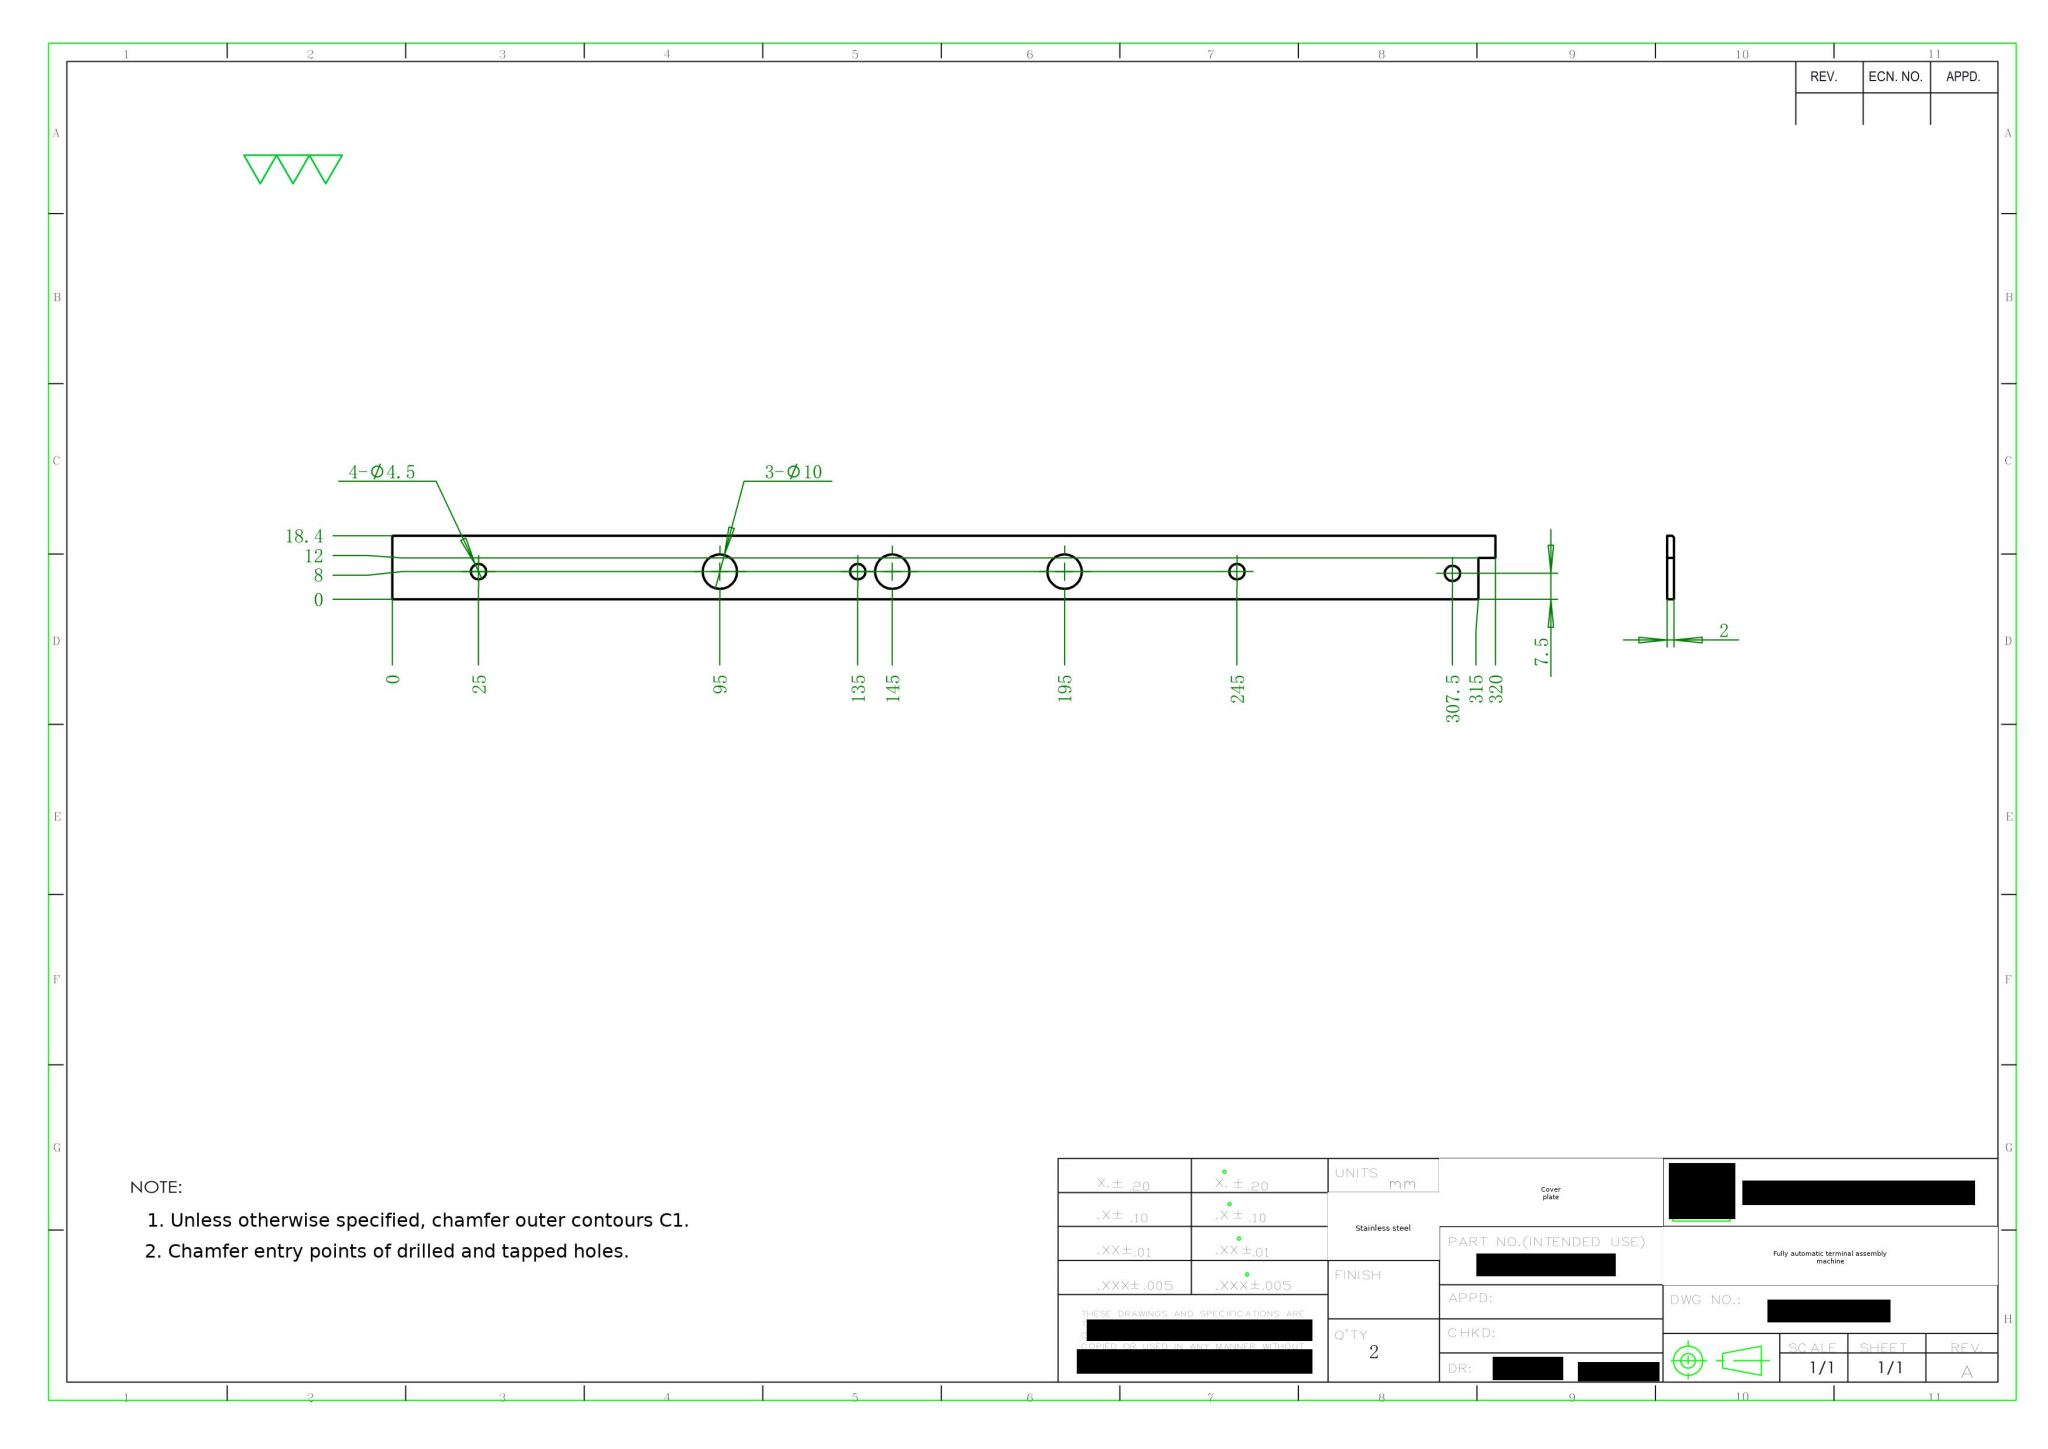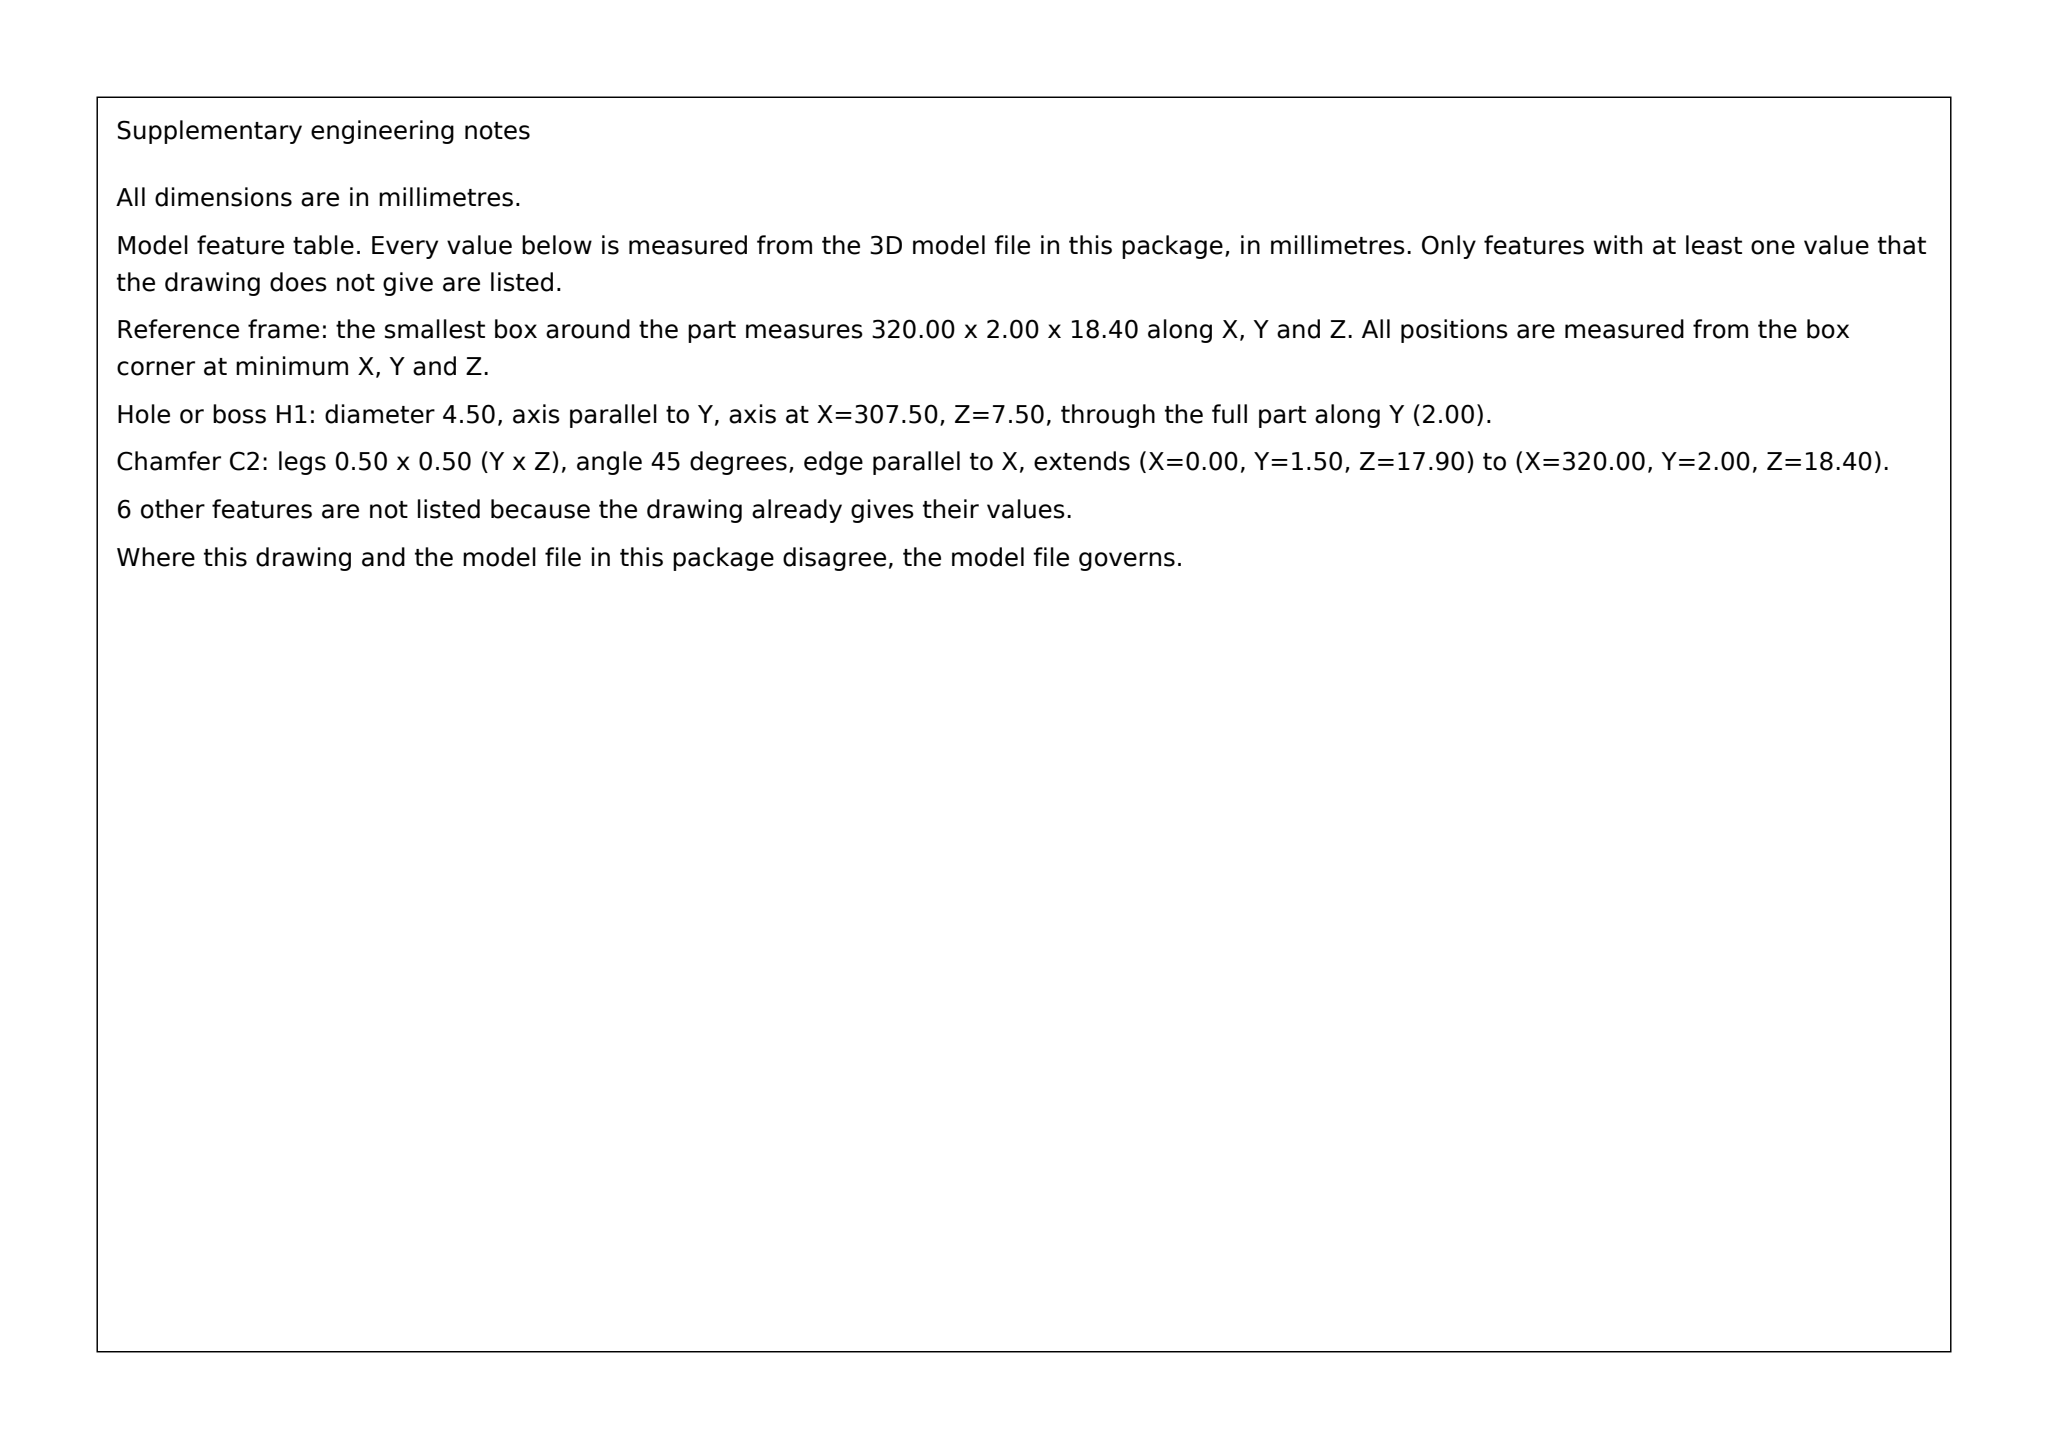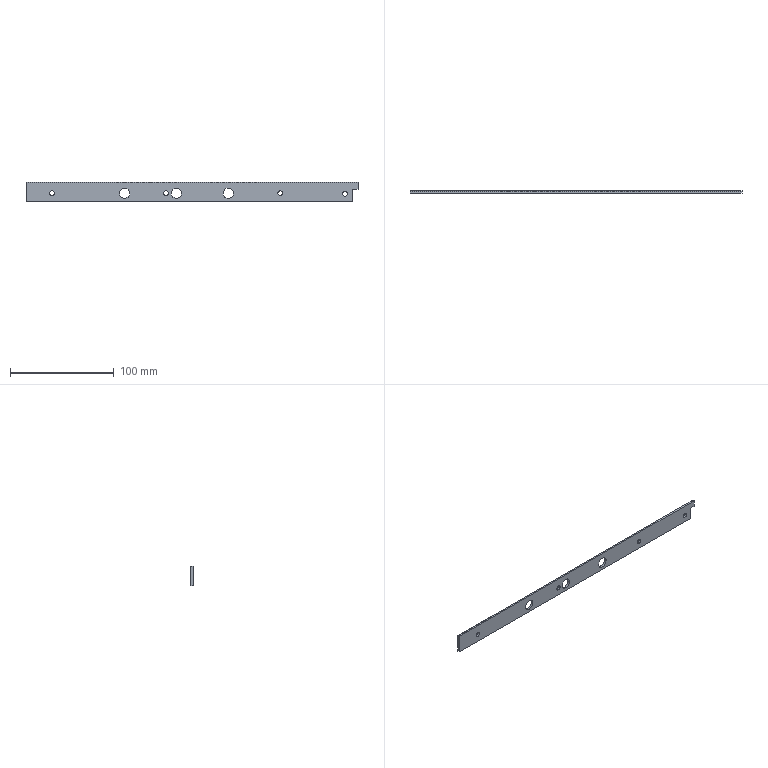Part | SolidWorks | mm | material Stainless steel | 1 solid | 23 faces | box 320 x 2 x 18.4 mm | volume 11018 mm3 | cylinder 14 | plane 9 | commonest cylinder face diameters 4.5 x8 10 x6
build123d program:
from build123d import *

# Parameters (mm, degrees)
SKETCH2_W                  = 320
SKETCH2_H                  = 18.4
BOSS_EXTRUDE1_DEPTH        = 2
CHAMFER1_SIZE              = 0.5
SKETCH8_W                  = 5
SKETCH8_H                  = 12
CUT_EXTRUDE2_DEPTH         = 161.277
F_4_5_4_5_DIAMETER_HOLE1_D = 4.5
F_10_0_10_DIAMETER_HOLE1_D = 10
F_4_5_4_5_DIAMETER_HOLE2_D = 4.5


with BuildPart() as part:
    # Sketch2 → Boss-Extrude1 (new body)
    with BuildSketch(Plane(origin=(0, 0, 0), x_dir=(1, 0, 0), z_dir=(0, 1, 0))):
        Rectangle(SKETCH2_W, SKETCH2_H)
    extrude(amount=BOSS_EXTRUDE1_DEPTH)

    # Chamfer1
    chamfer1_edges = [part.edges().sort_by_distance(p)[0] for p in [
        (0, 2, 9.2),
    ]]
    chamfer(chamfer1_edges, length=CHAMFER1_SIZE)

    # Sketch8 → Cut-Extrude2 (cut, through all)
    with BuildSketch(Plane(origin=(0, 2, 0), x_dir=(1, 0, 0), z_dir=(0, 1, 0))):
        with Locations((157.5, 3.2)):
            Rectangle(SKETCH8_W, SKETCH8_H)
    extrude(amount=-CUT_EXTRUDE2_DEPTH, mode=Mode.SUBTRACT)

    # 4.5 _4.5_ Diameter Hole1 (through all)
    with Locations(Plane(origin=(0, 2, 0), x_dir=(1, 0, 0), z_dir=(0, 1, 0))):
        with Locations((147.5, 1.7)):
            Hole(F_4_5_4_5_DIAMETER_HOLE1_D / 2)

    # 10.0 _10_ Diameter Hole1 (through all)
    with Locations(Plane(origin=(0, 2, 0), x_dir=(1, 0, 0), z_dir=(0, 1, 0))):
        with Locations((35, 1.2), (-15, 1.2), (-65, 1.2)):
            Hole(F_10_0_10_DIAMETER_HOLE1_D / 2)

    # 4.5 _4.5_ Diameter Hole2 (through all)
    with Locations(Plane(origin=(0, 0, 0), x_dir=(-1, 0, 0), z_dir=(0, -1, 0))):
        with Locations((135, 1.2), (25, 1.2), (-85, 1.2)):
            Hole(F_4_5_4_5_DIAMETER_HOLE2_D / 2)


solid = part.part
STEP:
#1=CARTESIAN_POINT('',(-135.,2.,1.05));
#2=VERTEX_POINT('',#1);
#3=CARTESIAN_POINT('',(-135.,2.,-3.45));
#4=VERTEX_POINT('',#3);
#5=CARTESIAN_POINT('',(-135.,2.,-1.2));
#6=DIRECTION('',(0.,-1.,0.));
#7=DIRECTION('',(0.,0.,-1.));
#8=AXIS2_PLACEMENT_3D('',#5,#6,#7);
#9=CIRCLE('',#8,2.25);
#10=EDGE_CURVE('',#2,#4,#9,.T.);
#11=ORIENTED_EDGE('',*,*,#10,.F.);
#12=CARTESIAN_POINT('',(-135.,0.,1.05));
#13=VERTEX_POINT('',#12);
#14=CARTESIAN_POINT('',(-135.,0.,1.05));
#15=DIRECTION('',(0.,-1.,0.));
#16=VECTOR('',#15,1000.);
#17=LINE('',#14,#16);
#18=EDGE_CURVE('',#2,#13,#17,.T.);
#19=ORIENTED_EDGE('',*,*,#18,.T.);
#20=CARTESIAN_POINT('',(-135.,0.,-3.45));
#21=VERTEX_POINT('',#20);
#22=CARTESIAN_POINT('',(-135.,0.,-1.2));
#23=DIRECTION('',(0.,-1.,0.));
#24=DIRECTION('',(0.,0.,-1.));
#25=AXIS2_PLACEMENT_3D('',#22,#23,#24);
#26=CIRCLE('',#25,2.25);
#27=EDGE_CURVE('',#13,#21,#26,.T.);
#28=ORIENTED_EDGE('',*,*,#27,.T.);
#29=CARTESIAN_POINT('',(-135.,0.,-3.45));
#30=DIRECTION('',(0.,-1.,0.));
#31=VECTOR('',#30,1000.);
#32=LINE('',#29,#31);
#33=EDGE_CURVE('',#4,#21,#32,.T.);
#34=ORIENTED_EDGE('',*,*,#33,.F.);
#35=EDGE_LOOP('',(#11,#19,#28,#34));
#36=FACE_OUTER_BOUND('',#35,.T.);
#37=CARTESIAN_POINT('',(-135.,0.,-1.2));
#38=DIRECTION('',(0.,-1.,0.));
#39=DIRECTION('',(0.,0.,-1.));
#40=AXIS2_PLACEMENT_3D('',#37,#38,#39);
#41=CYLINDRICAL_SURFACE('',#40,2.25);
#42=ADVANCED_FACE('',(#36),#41,.F.);
#43=CARTESIAN_POINT('',(-25.,2.,1.05));
#44=VERTEX_POINT('',#43);
#45=CARTESIAN_POINT('',(-25.,2.,-3.45));
#46=VERTEX_POINT('',#45);
#47=CARTESIAN_POINT('',(-25.,2.,-1.2));
#48=DIRECTION('',(0.,-1.,0.));
#49=DIRECTION('',(0.,0.,-1.));
#50=AXIS2_PLACEMENT_3D('',#47,#48,#49);
#51=CIRCLE('',#50,2.25);
#52=EDGE_CURVE('',#44,#46,#51,.T.);
#53=ORIENTED_EDGE('',*,*,#52,.F.);
#54=CARTESIAN_POINT('',(-25.,0.,1.05));
#55=VERTEX_POINT('',#54);
#56=CARTESIAN_POINT('',(-25.,0.,1.05));
#57=DIRECTION('',(0.,-1.,0.));
#58=VECTOR('',#57,1000.);
#59=LINE('',#56,#58);
#60=EDGE_CURVE('',#44,#55,#59,.T.);
#61=ORIENTED_EDGE('',*,*,#60,.T.);
#62=CARTESIAN_POINT('',(-25.,0.,-3.45));
#63=VERTEX_POINT('',#62);
#64=CARTESIAN_POINT('',(-25.,0.,-1.2));
#65=DIRECTION('',(0.,-1.,0.));
#66=DIRECTION('',(0.,0.,-1.));
#67=AXIS2_PLACEMENT_3D('',#64,#65,#66);
#68=CIRCLE('',#67,2.25);
#69=EDGE_CURVE('',#55,#63,#68,.T.);
#70=ORIENTED_EDGE('',*,*,#69,.T.);
#71=CARTESIAN_POINT('',(-25.,0.,-3.45));
#72=DIRECTION('',(0.,-1.,0.));
#73=VECTOR('',#72,1000.);
#74=LINE('',#71,#73);
#75=EDGE_CURVE('',#46,#63,#74,.T.);
#76=ORIENTED_EDGE('',*,*,#75,.F.);
#77=EDGE_LOOP('',(#53,#61,#70,#76));
#78=FACE_OUTER_BOUND('',#77,.T.);
#79=CARTESIAN_POINT('',(-25.,0.,-1.2));
#80=DIRECTION('',(0.,-1.,0.));
#81=DIRECTION('',(0.,0.,-1.));
#82=AXIS2_PLACEMENT_3D('',#79,#80,#81);
#83=CYLINDRICAL_SURFACE('',#82,2.25);
#84=ADVANCED_FACE('',(#78),#83,.F.);
#85=CARTESIAN_POINT('',(85.,2.,1.05));
#86=VERTEX_POINT('',#85);
#87=CARTESIAN_POINT('',(85.,2.,-3.45));
#88=VERTEX_POINT('',#87);
#89=CARTESIAN_POINT('',(85.,2.,-1.2));
#90=DIRECTION('',(0.,-1.,0.));
#91=DIRECTION('',(0.,0.,-1.));
#92=AXIS2_PLACEMENT_3D('',#89,#90,#91);
#93=CIRCLE('',#92,2.25);
#94=EDGE_CURVE('',#86,#88,#93,.T.);
#95=ORIENTED_EDGE('',*,*,#94,.F.);
#96=CARTESIAN_POINT('',(85.,0.,1.05));
#97=VERTEX_POINT('',#96);
#98=CARTESIAN_POINT('',(85.,0.,1.05));
#99=DIRECTION('',(0.,-1.,0.));
#100=VECTOR('',#99,1000.);
#101=LINE('',#98,#100);
#102=EDGE_CURVE('',#86,#97,#101,.T.);
#103=ORIENTED_EDGE('',*,*,#102,.T.);
#104=CARTESIAN_POINT('',(85.,0.,-3.45));
#105=VERTEX_POINT('',#104);
#106=CARTESIAN_POINT('',(85.,0.,-1.2));
#107=DIRECTION('',(0.,-1.,0.));
#108=DIRECTION('',(0.,0.,-1.));
#109=AXIS2_PLACEMENT_3D('',#106,#107,#108);
#110=CIRCLE('',#109,2.25);
#111=EDGE_CURVE('',#97,#105,#110,.T.);
#112=ORIENTED_EDGE('',*,*,#111,.T.);
#113=CARTESIAN_POINT('',(85.,0.,-3.45));
#114=DIRECTION('',(0.,-1.,0.));
#115=VECTOR('',#114,1000.);
#116=LINE('',#113,#115);
#117=EDGE_CURVE('',#88,#105,#116,.T.);
#118=ORIENTED_EDGE('',*,*,#117,.F.);
#119=EDGE_LOOP('',(#95,#103,#112,#118));
#120=FACE_OUTER_BOUND('',#119,.T.);
#121=CARTESIAN_POINT('',(85.,0.,-1.2));
#122=DIRECTION('',(0.,-1.,0.));
#123=DIRECTION('',(0.,0.,-1.));
#124=AXIS2_PLACEMENT_3D('',#121,#122,#123);
#125=CYLINDRICAL_SURFACE('',#124,2.25);
#126=ADVANCED_FACE('',(#120),#125,.F.);
#127=CARTESIAN_POINT('',(35.,0.,-6.2));
#128=VERTEX_POINT('',#127);
#129=CARTESIAN_POINT('',(35.,0.,3.8));
#130=VERTEX_POINT('',#129);
#131=CARTESIAN_POINT('',(35.,0.,-1.2));
#132=DIRECTION('',(0.,1.,0.));
#133=DIRECTION('',(0.,0.,1.));
#134=AXIS2_PLACEMENT_3D('',#131,#132,#133);
#135=CIRCLE('',#134,5.);
#136=EDGE_CURVE('',#128,#130,#135,.T.);
#137=ORIENTED_EDGE('',*,*,#136,.F.);
#138=CARTESIAN_POINT('',(35.,2.,-6.2));
#139=VERTEX_POINT('',#138);
#140=CARTESIAN_POINT('',(35.,2.,-6.2));
#141=DIRECTION('',(0.,1.,0.));
#142=VECTOR('',#141,1000.);
#143=LINE('',#140,#142);
#144=EDGE_CURVE('',#128,#139,#143,.T.);
#145=ORIENTED_EDGE('',*,*,#144,.T.);
#146=CARTESIAN_POINT('',(35.,2.,3.8));
#147=VERTEX_POINT('',#146);
#148=CARTESIAN_POINT('',(35.,2.,-1.2));
#149=DIRECTION('',(0.,1.,0.));
#150=DIRECTION('',(0.,0.,1.));
#151=AXIS2_PLACEMENT_3D('',#148,#149,#150);
#152=CIRCLE('',#151,5.);
#153=EDGE_CURVE('',#139,#147,#152,.T.);
#154=ORIENTED_EDGE('',*,*,#153,.T.);
#155=CARTESIAN_POINT('',(35.,2.,3.8));
#156=DIRECTION('',(0.,1.,0.));
#157=VECTOR('',#156,1000.);
#158=LINE('',#155,#157);
#159=EDGE_CURVE('',#130,#147,#158,.T.);
#160=ORIENTED_EDGE('',*,*,#159,.F.);
#161=EDGE_LOOP('',(#137,#145,#154,#160));
#162=FACE_OUTER_BOUND('',#161,.T.);
#163=CARTESIAN_POINT('',(35.,2.,-1.2));
#164=DIRECTION('',(0.,1.,0.));
#165=DIRECTION('',(0.,0.,1.));
#166=AXIS2_PLACEMENT_3D('',#163,#164,#165);
#167=CYLINDRICAL_SURFACE('',#166,5.);
#168=ADVANCED_FACE('',(#162),#167,.F.);
#169=CARTESIAN_POINT('',(-15.,0.,-6.2));
#170=VERTEX_POINT('',#169);
#171=CARTESIAN_POINT('',(-15.,0.,3.8));
#172=VERTEX_POINT('',#171);
#173=CARTESIAN_POINT('',(-15.,0.,-1.2));
#174=DIRECTION('',(0.,1.,0.));
#175=DIRECTION('',(0.,0.,1.));
#176=AXIS2_PLACEMENT_3D('',#173,#174,#175);
#177=CIRCLE('',#176,5.);
#178=EDGE_CURVE('',#170,#172,#177,.T.);
#179=ORIENTED_EDGE('',*,*,#178,.F.);
#180=CARTESIAN_POINT('',(-15.,2.,-6.2));
#181=VERTEX_POINT('',#180);
#182=CARTESIAN_POINT('',(-15.,2.,-6.2));
#183=DIRECTION('',(0.,1.,0.));
#184=VECTOR('',#183,1000.);
#185=LINE('',#182,#184);
#186=EDGE_CURVE('',#170,#181,#185,.T.);
#187=ORIENTED_EDGE('',*,*,#186,.T.);
#188=CARTESIAN_POINT('',(-15.,2.,3.8));
#189=VERTEX_POINT('',#188);
#190=CARTESIAN_POINT('',(-15.,2.,-1.2));
#191=DIRECTION('',(0.,1.,0.));
#192=DIRECTION('',(0.,0.,1.));
#193=AXIS2_PLACEMENT_3D('',#190,#191,#192);
#194=CIRCLE('',#193,5.);
#195=EDGE_CURVE('',#181,#189,#194,.T.);
#196=ORIENTED_EDGE('',*,*,#195,.T.);
#197=CARTESIAN_POINT('',(-15.,2.,3.8));
#198=DIRECTION('',(0.,1.,0.));
#199=VECTOR('',#198,1000.);
#200=LINE('',#197,#199);
#201=EDGE_CURVE('',#172,#189,#200,.T.);
#202=ORIENTED_EDGE('',*,*,#201,.F.);
#203=EDGE_LOOP('',(#179,#187,#196,#202));
#204=FACE_OUTER_BOUND('',#203,.T.);
#205=CARTESIAN_POINT('',(-15.,2.,-1.2));
#206=DIRECTION('',(0.,1.,0.));
#207=DIRECTION('',(0.,0.,1.));
#208=AXIS2_PLACEMENT_3D('',#205,#206,#207);
#209=CYLINDRICAL_SURFACE('',#208,5.);
#210=ADVANCED_FACE('',(#204),#209,.F.);
#211=CARTESIAN_POINT('',(-65.,0.,-6.2));
#212=VERTEX_POINT('',#211);
#213=CARTESIAN_POINT('',(-65.,0.,3.8));
#214=VERTEX_POINT('',#213);
#215=CARTESIAN_POINT('',(-65.,0.,-1.2));
#216=DIRECTION('',(0.,1.,0.));
#217=DIRECTION('',(0.,0.,1.));
#218=AXIS2_PLACEMENT_3D('',#215,#216,#217);
#219=CIRCLE('',#218,5.);
#220=EDGE_CURVE('',#212,#214,#219,.T.);
#221=ORIENTED_EDGE('',*,*,#220,.F.);
#222=CARTESIAN_POINT('',(-65.,2.,-6.2));
#223=VERTEX_POINT('',#222);
#224=CARTESIAN_POINT('',(-65.,2.,-6.2));
#225=DIRECTION('',(0.,1.,0.));
#226=VECTOR('',#225,1000.);
#227=LINE('',#224,#226);
#228=EDGE_CURVE('',#212,#223,#227,.T.);
#229=ORIENTED_EDGE('',*,*,#228,.T.);
#230=CARTESIAN_POINT('',(-65.,2.,3.8));
#231=VERTEX_POINT('',#230);
#232=CARTESIAN_POINT('',(-65.,2.,-1.2));
#233=DIRECTION('',(0.,1.,0.));
#234=DIRECTION('',(0.,0.,1.));
#235=AXIS2_PLACEMENT_3D('',#232,#233,#234);
#236=CIRCLE('',#235,5.);
#237=EDGE_CURVE('',#223,#231,#236,.T.);
#238=ORIENTED_EDGE('',*,*,#237,.T.);
#239=CARTESIAN_POINT('',(-65.,2.,3.8));
#240=DIRECTION('',(0.,1.,0.));
#241=VECTOR('',#240,1000.);
#242=LINE('',#239,#241);
#243=EDGE_CURVE('',#214,#231,#242,.T.);
#244=ORIENTED_EDGE('',*,*,#243,.F.);
#245=EDGE_LOOP('',(#221,#229,#238,#244));
#246=FACE_OUTER_BOUND('',#245,.T.);
#247=CARTESIAN_POINT('',(-65.,2.,-1.2));
#248=DIRECTION('',(0.,1.,0.));
#249=DIRECTION('',(0.,0.,1.));
#250=AXIS2_PLACEMENT_3D('',#247,#248,#249);
#251=CYLINDRICAL_SURFACE('',#250,5.);
#252=ADVANCED_FACE('',(#246),#251,.F.);
#253=CARTESIAN_POINT('',(147.5,0.,-3.95));
#254=VERTEX_POINT('',#253);
#255=CARTESIAN_POINT('',(147.5,0.,0.55));
#256=VERTEX_POINT('',#255);
#257=CARTESIAN_POINT('',(147.5,0.,-1.7));
#258=DIRECTION('',(0.,1.,0.));
#259=DIRECTION('',(0.,0.,1.));
#260=AXIS2_PLACEMENT_3D('',#257,#258,#259);
#261=CIRCLE('',#260,2.25);
#262=EDGE_CURVE('',#254,#256,#261,.T.);
#263=ORIENTED_EDGE('',*,*,#262,.F.);
#264=CARTESIAN_POINT('',(147.5,2.,-3.95));
#265=VERTEX_POINT('',#264);
#266=CARTESIAN_POINT('',(147.5,2.,-3.95));
#267=DIRECTION('',(0.,1.,0.));
#268=VECTOR('',#267,1000.);
#269=LINE('',#266,#268);
#270=EDGE_CURVE('',#254,#265,#269,.T.);
#271=ORIENTED_EDGE('',*,*,#270,.T.);
#272=CARTESIAN_POINT('',(147.5,2.,0.55));
#273=VERTEX_POINT('',#272);
#274=CARTESIAN_POINT('',(147.5,2.,-1.7));
#275=DIRECTION('',(0.,1.,0.));
#276=DIRECTION('',(0.,0.,1.));
#277=AXIS2_PLACEMENT_3D('',#274,#275,#276);
#278=CIRCLE('',#277,2.25);
#279=EDGE_CURVE('',#265,#273,#278,.T.);
#280=ORIENTED_EDGE('',*,*,#279,.T.);
#281=CARTESIAN_POINT('',(147.5,2.,0.55));
#282=DIRECTION('',(0.,1.,0.));
#283=VECTOR('',#282,1000.);
#284=LINE('',#281,#283);
#285=EDGE_CURVE('',#256,#273,#284,.T.);
#286=ORIENTED_EDGE('',*,*,#285,.F.);
#287=EDGE_LOOP('',(#263,#271,#280,#286));
#288=FACE_OUTER_BOUND('',#287,.T.);
#289=CARTESIAN_POINT('',(147.5,2.,-1.7));
#290=DIRECTION('',(0.,1.,0.));
#291=DIRECTION('',(0.,0.,1.));
#292=AXIS2_PLACEMENT_3D('',#289,#290,#291);
#293=CYLINDRICAL_SURFACE('',#292,2.25);
#294=ADVANCED_FACE('',(#288),#293,.F.);
#295=CARTESIAN_POINT('',(-135.,0.,-1.2));
#296=DIRECTION('',(0.,-1.,0.));
#297=DIRECTION('',(0.,0.,-1.));
#298=AXIS2_PLACEMENT_3D('',#295,#296,#297);
#299=CIRCLE('',#298,2.25);
#300=EDGE_CURVE('',#21,#13,#299,.T.);
#301=ORIENTED_EDGE('',*,*,#300,.F.);
#302=ORIENTED_EDGE('',*,*,#27,.F.);
#303=EDGE_LOOP('',(#301,#302));
#304=FACE_BOUND('',#303,.T.);
#305=CARTESIAN_POINT('',(-25.,0.,-1.2));
#306=DIRECTION('',(0.,-1.,0.));
#307=DIRECTION('',(0.,0.,-1.));
#308=AXIS2_PLACEMENT_3D('',#305,#306,#307);
#309=CIRCLE('',#308,2.25);
#310=EDGE_CURVE('',#63,#55,#309,.T.);
#311=ORIENTED_EDGE('',*,*,#310,.F.);
#312=ORIENTED_EDGE('',*,*,#69,.F.);
#313=EDGE_LOOP('',(#311,#312));
#314=FACE_BOUND('',#313,.T.);
#315=CARTESIAN_POINT('',(85.,0.,-1.2));
#316=DIRECTION('',(0.,-1.,0.));
#317=DIRECTION('',(0.,0.,-1.));
#318=AXIS2_PLACEMENT_3D('',#315,#316,#317);
#319=CIRCLE('',#318,2.25);
#320=EDGE_CURVE('',#105,#97,#319,.T.);
#321=ORIENTED_EDGE('',*,*,#320,.F.);
#322=ORIENTED_EDGE('',*,*,#111,.F.);
#323=EDGE_LOOP('',(#321,#322));
#324=FACE_BOUND('',#323,.T.);
#325=CARTESIAN_POINT('',(155.,0.,2.8));
#326=VERTEX_POINT('',#325);
#327=CARTESIAN_POINT('',(160.,0.,2.8));
#328=VERTEX_POINT('',#327);
#329=CARTESIAN_POINT('',(160.,0.,2.8));
#330=DIRECTION('',(1.,0.,-0.));
#331=VECTOR('',#330,1000.);
#332=LINE('',#329,#331);
#333=EDGE_CURVE('',#326,#328,#332,.T.);
#334=ORIENTED_EDGE('',*,*,#333,.T.);
#335=CARTESIAN_POINT('',(160.,0.,9.2));
#336=VERTEX_POINT('',#335);
#337=CARTESIAN_POINT('',(160.,0.,9.2));
#338=DIRECTION('',(0.,0.,-1.));
#339=VECTOR('',#338,1000.);
#340=LINE('',#337,#339);
#341=EDGE_CURVE('',#336,#328,#340,.T.);
#342=ORIENTED_EDGE('',*,*,#341,.F.);
#343=CARTESIAN_POINT('',(-160.,0.,9.2));
#344=VERTEX_POINT('',#343);
#345=CARTESIAN_POINT('',(-160.,0.,9.2));
#346=DIRECTION('',(1.,0.,0.));
#347=VECTOR('',#346,1000.);
#348=LINE('',#345,#347);
#349=EDGE_CURVE('',#344,#336,#348,.T.);
#350=ORIENTED_EDGE('',*,*,#349,.F.);
#351=CARTESIAN_POINT('',(-160.,0.,-9.2));
#352=VERTEX_POINT('',#351);
#353=CARTESIAN_POINT('',(-160.,0.,9.2));
#354=DIRECTION('',(0.,0.,1.));
#355=VECTOR('',#354,1000.);
#356=LINE('',#353,#355);
#357=EDGE_CURVE('',#352,#344,#356,.T.);
#358=ORIENTED_EDGE('',*,*,#357,.F.);
#359=CARTESIAN_POINT('',(155.,0.,-9.2));
#360=VERTEX_POINT('',#359);
#361=CARTESIAN_POINT('',(-160.,0.,-9.2));
#362=DIRECTION('',(-1.,0.,0.));
#363=VECTOR('',#362,1000.);
#364=LINE('',#361,#363);
#365=EDGE_CURVE('',#360,#352,#364,.T.);
#366=ORIENTED_EDGE('',*,*,#365,.F.);
#367=CARTESIAN_POINT('',(155.,0.,-9.2));
#368=DIRECTION('',(0.,0.,1.));
#369=VECTOR('',#368,1000.);
#370=LINE('',#367,#369);
#371=EDGE_CURVE('',#360,#326,#370,.T.);
#372=ORIENTED_EDGE('',*,*,#371,.T.);
#373=EDGE_LOOP('',(#334,#342,#350,#358,#366,#372));
#374=FACE_OUTER_BOUND('',#373,.T.);
#375=CARTESIAN_POINT('',(147.5,0.,-1.7));
#376=DIRECTION('',(0.,1.,0.));
#377=DIRECTION('',(0.,0.,1.));
#378=AXIS2_PLACEMENT_3D('',#375,#376,#377);
#379=CIRCLE('',#378,2.25);
#380=EDGE_CURVE('',#256,#254,#379,.T.);
#381=ORIENTED_EDGE('',*,*,#380,.T.);
#382=ORIENTED_EDGE('',*,*,#262,.T.);
#383=EDGE_LOOP('',(#381,#382));
#384=FACE_BOUND('',#383,.T.);
#385=CARTESIAN_POINT('',(-65.,0.,-1.2));
#386=DIRECTION('',(0.,1.,0.));
#387=DIRECTION('',(0.,0.,1.));
#388=AXIS2_PLACEMENT_3D('',#385,#386,#387);
#389=CIRCLE('',#388,5.);
#390=EDGE_CURVE('',#214,#212,#389,.T.);
#391=ORIENTED_EDGE('',*,*,#390,.T.);
#392=ORIENTED_EDGE('',*,*,#220,.T.);
#393=EDGE_LOOP('',(#391,#392));
#394=FACE_BOUND('',#393,.T.);
#395=CARTESIAN_POINT('',(-15.,0.,-1.2));
#396=DIRECTION('',(0.,1.,0.));
#397=DIRECTION('',(0.,0.,1.));
#398=AXIS2_PLACEMENT_3D('',#395,#396,#397);
#399=CIRCLE('',#398,5.);
#400=EDGE_CURVE('',#172,#170,#399,.T.);
#401=ORIENTED_EDGE('',*,*,#400,.T.);
#402=ORIENTED_EDGE('',*,*,#178,.T.);
#403=EDGE_LOOP('',(#401,#402));
#404=FACE_BOUND('',#403,.T.);
#405=CARTESIAN_POINT('',(35.,0.,-1.2));
#406=DIRECTION('',(0.,1.,0.));
#407=DIRECTION('',(0.,0.,1.));
#408=AXIS2_PLACEMENT_3D('',#405,#406,#407);
#409=CIRCLE('',#408,5.);
#410=EDGE_CURVE('',#130,#128,#409,.T.);
#411=ORIENTED_EDGE('',*,*,#410,.T.);
#412=ORIENTED_EDGE('',*,*,#136,.T.);
#413=EDGE_LOOP('',(#411,#412));
#414=FACE_BOUND('',#413,.T.);
#415=CARTESIAN_POINT('',(0.,0.,0.));
#416=DIRECTION('',(0.,-1.,0.));
#417=DIRECTION('',(0.,0.,-1.));
#418=AXIS2_PLACEMENT_3D('',#415,#416,#417);
#419=PLANE('',#418);
#420=ADVANCED_FACE('',(#304,#314,#324,#374,#384,#394,#404,#414),#419,.T.);
#421=ORIENTED_EDGE('',*,*,#341,.T.);
#422=CARTESIAN_POINT('',(160.,2.,2.8));
#423=VERTEX_POINT('',#422);
#424=CARTESIAN_POINT('',(160.,0.,2.8));
#425=DIRECTION('',(0.,1.,0.));
#426=VECTOR('',#425,1000.);
#427=LINE('',#424,#426);
#428=EDGE_CURVE('',#328,#423,#427,.T.);
#429=ORIENTED_EDGE('',*,*,#428,.T.);
#430=CARTESIAN_POINT('',(160.,2.,8.7));
#431=VERTEX_POINT('',#430);
#432=CARTESIAN_POINT('',(160.,2.,9.2));
#433=DIRECTION('',(0.,0.,-1.));
#434=VECTOR('',#433,1000.);
#435=LINE('',#432,#434);
#436=EDGE_CURVE('',#431,#423,#435,.T.);
#437=ORIENTED_EDGE('',*,*,#436,.F.);
#438=CARTESIAN_POINT('',(160.,1.5,9.2));
#439=VERTEX_POINT('',#438);
#440=CARTESIAN_POINT('',(160.,2.,8.7));
#441=DIRECTION('',(0.,-0.7071,0.7071));
#442=VECTOR('',#441,1000.);
#443=LINE('',#440,#442);
#444=EDGE_CURVE('',#431,#439,#443,.T.);
#445=ORIENTED_EDGE('',*,*,#444,.T.);
#446=CARTESIAN_POINT('',(160.,2.,9.2));
#447=DIRECTION('',(0.,-1.,0.));
#448=VECTOR('',#447,1000.);
#449=LINE('',#446,#448);
#450=EDGE_CURVE('',#439,#336,#449,.T.);
#451=ORIENTED_EDGE('',*,*,#450,.T.);
#452=EDGE_LOOP('',(#421,#429,#437,#445,#451));
#453=FACE_OUTER_BOUND('',#452,.T.);
#454=CARTESIAN_POINT('',(160.,2.,9.2));
#455=DIRECTION('',(-1.,0.,0.));
#456=DIRECTION('',(0.,0.,1.));
#457=AXIS2_PLACEMENT_3D('',#454,#455,#456);
#458=PLANE('',#457);
#459=ADVANCED_FACE('',(#453),#458,.F.);
#460=CARTESIAN_POINT('',(155.,2.,-9.2));
#461=VERTEX_POINT('',#460);
#462=CARTESIAN_POINT('',(-160.,2.,-9.2));
#463=VERTEX_POINT('',#462);
#464=CARTESIAN_POINT('',(-160.,2.,-9.2));
#465=DIRECTION('',(-1.,0.,0.));
#466=VECTOR('',#465,1000.);
#467=LINE('',#464,#466);
#468=EDGE_CURVE('',#461,#463,#467,.T.);
#469=ORIENTED_EDGE('',*,*,#468,.F.);
#470=CARTESIAN_POINT('',(155.,0.,-9.2));
#471=DIRECTION('',(0.,1.,0.));
#472=VECTOR('',#471,1000.);
#473=LINE('',#470,#472);
#474=EDGE_CURVE('',#360,#461,#473,.T.);
#475=ORIENTED_EDGE('',*,*,#474,.F.);
#476=ORIENTED_EDGE('',*,*,#365,.T.);
#477=CARTESIAN_POINT('',(-160.,2.,-9.2));
#478=DIRECTION('',(0.,-1.,0.));
#479=VECTOR('',#478,1000.);
#480=LINE('',#477,#479);
#481=EDGE_CURVE('',#463,#352,#480,.T.);
#482=ORIENTED_EDGE('',*,*,#481,.F.);
#483=EDGE_LOOP('',(#469,#475,#476,#482));
#484=FACE_OUTER_BOUND('',#483,.T.);
#485=CARTESIAN_POINT('',(-160.,2.,-9.2));
#486=DIRECTION('',(0.,0.,1.));
#487=DIRECTION('',(1.,0.,0.));
#488=AXIS2_PLACEMENT_3D('',#485,#486,#487);
#489=PLANE('',#488);
#490=ADVANCED_FACE('',(#484),#489,.F.);
#491=CARTESIAN_POINT('',(-160.,1.5,9.2));
#492=VERTEX_POINT('',#491);
#493=CARTESIAN_POINT('',(-160.,2.,9.2));
#494=DIRECTION('',(0.,-1.,0.));
#495=VECTOR('',#494,1000.);
#496=LINE('',#493,#495);
#497=EDGE_CURVE('',#492,#344,#496,.T.);
#498=ORIENTED_EDGE('',*,*,#497,.F.);
#499=CARTESIAN_POINT('',(-160.,2.,8.7));
#500=VERTEX_POINT('',#499);
#501=CARTESIAN_POINT('',(-160.,2.,8.7));
#502=DIRECTION('',(0.,0.7071,-0.7071));
#503=VECTOR('',#502,1000.);
#504=LINE('',#501,#503);
#505=EDGE_CURVE('',#492,#500,#504,.T.);
#506=ORIENTED_EDGE('',*,*,#505,.T.);
#507=CARTESIAN_POINT('',(-160.,2.,9.2));
#508=DIRECTION('',(0.,0.,1.));
#509=VECTOR('',#508,1000.);
#510=LINE('',#507,#509);
#511=EDGE_CURVE('',#463,#500,#510,.T.);
#512=ORIENTED_EDGE('',*,*,#511,.F.);
#513=ORIENTED_EDGE('',*,*,#481,.T.);
#514=ORIENTED_EDGE('',*,*,#357,.T.);
#515=EDGE_LOOP('',(#498,#506,#512,#513,#514));
#516=FACE_OUTER_BOUND('',#515,.T.);
#517=CARTESIAN_POINT('',(-160.,2.,9.2));
#518=DIRECTION('',(1.,0.,0.));
#519=DIRECTION('',(0.,0.,-1.));
#520=AXIS2_PLACEMENT_3D('',#517,#518,#519);
#521=PLANE('',#520);
#522=ADVANCED_FACE('',(#516),#521,.F.);
#523=ORIENTED_EDGE('',*,*,#450,.F.);
#524=CARTESIAN_POINT('',(-160.,1.5,9.2));
#525=DIRECTION('',(-1.,0.,0.));
#526=VECTOR('',#525,1000.);
#527=LINE('',#524,#526);
#528=EDGE_CURVE('',#439,#492,#527,.T.);
#529=ORIENTED_EDGE('',*,*,#528,.T.);
#530=ORIENTED_EDGE('',*,*,#497,.T.);
#531=ORIENTED_EDGE('',*,*,#349,.T.);
#532=EDGE_LOOP('',(#523,#529,#530,#531));
#533=FACE_OUTER_BOUND('',#532,.T.);
#534=CARTESIAN_POINT('',(-160.,2.,9.2));
#535=DIRECTION('',(0.,0.,-1.));
#536=DIRECTION('',(-1.,0.,0.));
#537=AXIS2_PLACEMENT_3D('',#534,#535,#536);
#538=PLANE('',#537);
#539=ADVANCED_FACE('',(#533),#538,.F.);
#540=CARTESIAN_POINT('',(-135.,2.,-1.2));
#541=DIRECTION('',(0.,-1.,0.));
#542=DIRECTION('',(0.,0.,-1.));
#543=AXIS2_PLACEMENT_3D('',#540,#541,#542);
#544=CIRCLE('',#543,2.25);
#545=EDGE_CURVE('',#4,#2,#544,.T.);
#546=ORIENTED_EDGE('',*,*,#545,.T.);
#547=ORIENTED_EDGE('',*,*,#10,.T.);
#548=EDGE_LOOP('',(#546,#547));
#549=FACE_BOUND('',#548,.T.);
#550=CARTESIAN_POINT('',(-25.,2.,-1.2));
#551=DIRECTION('',(0.,-1.,0.));
#552=DIRECTION('',(0.,0.,-1.));
#553=AXIS2_PLACEMENT_3D('',#550,#551,#552);
#554=CIRCLE('',#553,2.25);
#555=EDGE_CURVE('',#46,#44,#554,.T.);
#556=ORIENTED_EDGE('',*,*,#555,.T.);
#557=ORIENTED_EDGE('',*,*,#52,.T.);
#558=EDGE_LOOP('',(#556,#557));
#559=FACE_BOUND('',#558,.T.);
#560=CARTESIAN_POINT('',(85.,2.,-1.2));
#561=DIRECTION('',(0.,-1.,0.));
#562=DIRECTION('',(0.,0.,-1.));
#563=AXIS2_PLACEMENT_3D('',#560,#561,#562);
#564=CIRCLE('',#563,2.25);
#565=EDGE_CURVE('',#88,#86,#564,.T.);
#566=ORIENTED_EDGE('',*,*,#565,.T.);
#567=ORIENTED_EDGE('',*,*,#94,.T.);
#568=EDGE_LOOP('',(#566,#567));
#569=FACE_BOUND('',#568,.T.);
#570=CARTESIAN_POINT('',(35.,2.,-1.2));
#571=DIRECTION('',(0.,1.,0.));
#572=DIRECTION('',(0.,0.,1.));
#573=AXIS2_PLACEMENT_3D('',#570,#571,#572);
#574=CIRCLE('',#573,5.);
#575=EDGE_CURVE('',#147,#139,#574,.T.);
#576=ORIENTED_EDGE('',*,*,#575,.F.);
#577=ORIENTED_EDGE('',*,*,#153,.F.);
#578=EDGE_LOOP('',(#576,#577));
#579=FACE_BOUND('',#578,.T.);
#580=CARTESIAN_POINT('',(-15.,2.,-1.2));
#581=DIRECTION('',(0.,1.,0.));
#582=DIRECTION('',(0.,0.,1.));
#583=AXIS2_PLACEMENT_3D('',#580,#581,#582);
#584=CIRCLE('',#583,5.);
#585=EDGE_CURVE('',#189,#181,#584,.T.);
#586=ORIENTED_EDGE('',*,*,#585,.F.);
#587=ORIENTED_EDGE('',*,*,#195,.F.);
#588=EDGE_LOOP('',(#586,#587));
#589=FACE_BOUND('',#588,.T.);
#590=CARTESIAN_POINT('',(-65.,2.,-1.2));
#591=DIRECTION('',(0.,1.,0.));
#592=DIRECTION('',(0.,0.,1.));
#593=AXIS2_PLACEMENT_3D('',#590,#591,#592);
#594=CIRCLE('',#593,5.);
#595=EDGE_CURVE('',#231,#223,#594,.T.);
#596=ORIENTED_EDGE('',*,*,#595,.F.);
#597=ORIENTED_EDGE('',*,*,#237,.F.);
#598=EDGE_LOOP('',(#596,#597));
#599=FACE_BOUND('',#598,.T.);
#600=CARTESIAN_POINT('',(147.5,2.,-1.7));
#601=DIRECTION('',(0.,1.,0.));
#602=DIRECTION('',(0.,0.,1.));
#603=AXIS2_PLACEMENT_3D('',#600,#601,#602);
#604=CIRCLE('',#603,2.25);
#605=EDGE_CURVE('',#273,#265,#604,.T.);
#606=ORIENTED_EDGE('',*,*,#605,.F.);
#607=ORIENTED_EDGE('',*,*,#279,.F.);
#608=EDGE_LOOP('',(#606,#607));
#609=FACE_BOUND('',#608,.T.);
#610=ORIENTED_EDGE('',*,*,#436,.T.);
#611=CARTESIAN_POINT('',(155.,2.,2.8));
#612=VERTEX_POINT('',#611);
#613=CARTESIAN_POINT('',(160.,2.,2.8));
#614=DIRECTION('',(1.,0.,-0.));
#615=VECTOR('',#614,1000.);
#616=LINE('',#613,#615);
#617=EDGE_CURVE('',#612,#423,#616,.T.);
#618=ORIENTED_EDGE('',*,*,#617,.F.);
#619=CARTESIAN_POINT('',(155.,2.,-9.2));
#620=DIRECTION('',(0.,0.,1.));
#621=VECTOR('',#620,1000.);
#622=LINE('',#619,#621);
#623=EDGE_CURVE('',#461,#612,#622,.T.);
#624=ORIENTED_EDGE('',*,*,#623,.F.);
#625=ORIENTED_EDGE('',*,*,#468,.T.);
#626=ORIENTED_EDGE('',*,*,#511,.T.);
#627=CARTESIAN_POINT('',(0.,2.,8.7));
#628=DIRECTION('',(1.,0.,0.));
#629=VECTOR('',#628,1000.);
#630=LINE('',#627,#629);
#631=EDGE_CURVE('',#500,#431,#630,.T.);
#632=ORIENTED_EDGE('',*,*,#631,.T.);
#633=EDGE_LOOP('',(#610,#618,#624,#625,#626,#632));
#634=FACE_OUTER_BOUND('',#633,.T.);
#635=CARTESIAN_POINT('',(0.,2.,0.));
#636=DIRECTION('',(0.,-1.,0.));
#637=DIRECTION('',(0.,0.,-1.));
#638=AXIS2_PLACEMENT_3D('',#635,#636,#637);
#639=PLANE('',#638);
#640=ADVANCED_FACE('',(#549,#559,#569,#579,#589,#599,#609,#634),#639,.F.);
#641=ORIENTED_EDGE('',*,*,#505,.F.);
#642=ORIENTED_EDGE('',*,*,#528,.F.);
#643=ORIENTED_EDGE('',*,*,#444,.F.);
#644=ORIENTED_EDGE('',*,*,#631,.F.);
#645=EDGE_LOOP('',(#641,#642,#643,#644));
#646=FACE_OUTER_BOUND('',#645,.T.);
#647=CARTESIAN_POINT('',(0.,2.,8.7));
#648=DIRECTION('',(0.,-0.7071,-0.7071));
#649=DIRECTION('',(1.,0.,0.));
#650=AXIS2_PLACEMENT_3D('',#647,#648,#649);
#651=PLANE('',#650);
#652=ADVANCED_FACE('',(#646),#651,.F.);
#653=ORIENTED_EDGE('',*,*,#617,.T.);
#654=ORIENTED_EDGE('',*,*,#428,.F.);
#655=ORIENTED_EDGE('',*,*,#333,.F.);
#656=CARTESIAN_POINT('',(155.,0.,2.8));
#657=DIRECTION('',(0.,1.,0.));
#658=VECTOR('',#657,1000.);
#659=LINE('',#656,#658);
#660=EDGE_CURVE('',#326,#612,#659,.T.);
#661=ORIENTED_EDGE('',*,*,#660,.T.);
#662=EDGE_LOOP('',(#653,#654,#655,#661));
#663=FACE_OUTER_BOUND('',#662,.T.);
#664=CARTESIAN_POINT('',(160.,0.,2.8));
#665=DIRECTION('',(0.,0.,1.));
#666=DIRECTION('',(1.,0.,-0.));
#667=AXIS2_PLACEMENT_3D('',#664,#665,#666);
#668=PLANE('',#667);
#669=ADVANCED_FACE('',(#663),#668,.F.);
#670=ORIENTED_EDGE('',*,*,#623,.T.);
#671=ORIENTED_EDGE('',*,*,#660,.F.);
#672=ORIENTED_EDGE('',*,*,#371,.F.);
#673=ORIENTED_EDGE('',*,*,#474,.T.);
#674=EDGE_LOOP('',(#670,#671,#672,#673));
#675=FACE_OUTER_BOUND('',#674,.T.);
#676=CARTESIAN_POINT('',(155.,0.,-9.2));
#677=DIRECTION('',(-1.,0.,0.));
#678=DIRECTION('',(0.,0.,1.));
#679=AXIS2_PLACEMENT_3D('',#676,#677,#678);
#680=PLANE('',#679);
#681=ADVANCED_FACE('',(#675),#680,.F.);
#682=ORIENTED_EDGE('',*,*,#270,.F.);
#683=ORIENTED_EDGE('',*,*,#380,.F.);
#684=ORIENTED_EDGE('',*,*,#285,.T.);
#685=ORIENTED_EDGE('',*,*,#605,.T.);
#686=EDGE_LOOP('',(#682,#683,#684,#685));
#687=FACE_OUTER_BOUND('',#686,.T.);
#688=CARTESIAN_POINT('',(147.5,2.,-1.7));
#689=DIRECTION('',(0.,1.,0.));
#690=DIRECTION('',(0.,0.,1.));
#691=AXIS2_PLACEMENT_3D('',#688,#689,#690);
#692=CYLINDRICAL_SURFACE('',#691,2.25);
#693=ADVANCED_FACE('',(#687),#692,.F.);
#694=ORIENTED_EDGE('',*,*,#228,.F.);
#695=ORIENTED_EDGE('',*,*,#390,.F.);
#696=ORIENTED_EDGE('',*,*,#243,.T.);
#697=ORIENTED_EDGE('',*,*,#595,.T.);
#698=EDGE_LOOP('',(#694,#695,#696,#697));
#699=FACE_OUTER_BOUND('',#698,.T.);
#700=CARTESIAN_POINT('',(-65.,2.,-1.2));
#701=DIRECTION('',(0.,1.,0.));
#702=DIRECTION('',(0.,0.,1.));
#703=AXIS2_PLACEMENT_3D('',#700,#701,#702);
#704=CYLINDRICAL_SURFACE('',#703,5.);
#705=ADVANCED_FACE('',(#699),#704,.F.);
#706=ORIENTED_EDGE('',*,*,#186,.F.);
#707=ORIENTED_EDGE('',*,*,#400,.F.);
#708=ORIENTED_EDGE('',*,*,#201,.T.);
#709=ORIENTED_EDGE('',*,*,#585,.T.);
#710=EDGE_LOOP('',(#706,#707,#708,#709));
#711=FACE_OUTER_BOUND('',#710,.T.);
#712=CARTESIAN_POINT('',(-15.,2.,-1.2));
#713=DIRECTION('',(0.,1.,0.));
#714=DIRECTION('',(0.,0.,1.));
#715=AXIS2_PLACEMENT_3D('',#712,#713,#714);
#716=CYLINDRICAL_SURFACE('',#715,5.);
#717=ADVANCED_FACE('',(#711),#716,.F.);
#718=ORIENTED_EDGE('',*,*,#144,.F.);
#719=ORIENTED_EDGE('',*,*,#410,.F.);
#720=ORIENTED_EDGE('',*,*,#159,.T.);
#721=ORIENTED_EDGE('',*,*,#575,.T.);
#722=EDGE_LOOP('',(#718,#719,#720,#721));
#723=FACE_OUTER_BOUND('',#722,.T.);
#724=CARTESIAN_POINT('',(35.,2.,-1.2));
#725=DIRECTION('',(0.,1.,0.));
#726=DIRECTION('',(0.,0.,1.));
#727=AXIS2_PLACEMENT_3D('',#724,#725,#726);
#728=CYLINDRICAL_SURFACE('',#727,5.);
#729=ADVANCED_FACE('',(#723),#728,.F.);
#730=ORIENTED_EDGE('',*,*,#102,.F.);
#731=ORIENTED_EDGE('',*,*,#565,.F.);
#732=ORIENTED_EDGE('',*,*,#117,.T.);
#733=ORIENTED_EDGE('',*,*,#320,.T.);
#734=EDGE_LOOP('',(#730,#731,#732,#733));
#735=FACE_OUTER_BOUND('',#734,.T.);
#736=CARTESIAN_POINT('',(85.,0.,-1.2));
#737=DIRECTION('',(0.,-1.,0.));
#738=DIRECTION('',(0.,0.,-1.));
#739=AXIS2_PLACEMENT_3D('',#736,#737,#738);
#740=CYLINDRICAL_SURFACE('',#739,2.25);
#741=ADVANCED_FACE('',(#735),#740,.F.);
#742=ORIENTED_EDGE('',*,*,#60,.F.);
#743=ORIENTED_EDGE('',*,*,#555,.F.);
#744=ORIENTED_EDGE('',*,*,#75,.T.);
#745=ORIENTED_EDGE('',*,*,#310,.T.);
#746=EDGE_LOOP('',(#742,#743,#744,#745));
#747=FACE_OUTER_BOUND('',#746,.T.);
#748=CARTESIAN_POINT('',(-25.,0.,-1.2));
#749=DIRECTION('',(0.,-1.,0.));
#750=DIRECTION('',(0.,0.,-1.));
#751=AXIS2_PLACEMENT_3D('',#748,#749,#750);
#752=CYLINDRICAL_SURFACE('',#751,2.25);
#753=ADVANCED_FACE('',(#747),#752,.F.);
#754=ORIENTED_EDGE('',*,*,#18,.F.);
#755=ORIENTED_EDGE('',*,*,#545,.F.);
#756=ORIENTED_EDGE('',*,*,#33,.T.);
#757=ORIENTED_EDGE('',*,*,#300,.T.);
#758=EDGE_LOOP('',(#754,#755,#756,#757));
#759=FACE_OUTER_BOUND('',#758,.T.);
#760=CARTESIAN_POINT('',(-135.,0.,-1.2));
#761=DIRECTION('',(0.,-1.,0.));
#762=DIRECTION('',(0.,0.,-1.));
#763=AXIS2_PLACEMENT_3D('',#760,#761,#762);
#764=CYLINDRICAL_SURFACE('',#763,2.25);
#765=ADVANCED_FACE('',(#759),#764,.F.);
#766=CLOSED_SHELL('',(#42,#84,#126,#168,#210,#252,#294,#420,#459,#490,#522,#539,#640,#652,#669,#681,#693,#705,#717,#729,#741,#753,#765));
#767=MANIFOLD_SOLID_BREP('',#766);
#768=CARTESIAN_POINT('',(0.,0.,0.));
#769=DIRECTION('',(0.,0.,1.));
#770=DIRECTION('',(1.,0.,0.));
#771=AXIS2_PLACEMENT_3D('',#768,#769,#770);
#772=(LENGTH_UNIT()NAMED_UNIT(*)SI_UNIT(.MILLI.,.METRE.));
#773=UNCERTAINTY_MEASURE_WITH_UNIT(LENGTH_MEASURE(0.00001),#772,'','');
#774=(NAMED_UNIT(*)PLANE_ANGLE_UNIT()SI_UNIT($,.RADIAN.));
#775=(NAMED_UNIT(*)SI_UNIT($,.STERADIAN.)SOLID_ANGLE_UNIT());
#776=(GEOMETRIC_REPRESENTATION_CONTEXT(3)GLOBAL_UNCERTAINTY_ASSIGNED_CONTEXT((#773))GLOBAL_UNIT_ASSIGNED_CONTEXT((#772,#774,#775))REPRESENTATION_CONTEXT('',''));
#777=ADVANCED_BREP_SHAPE_REPRESENTATION('',(#767,#771),#776);